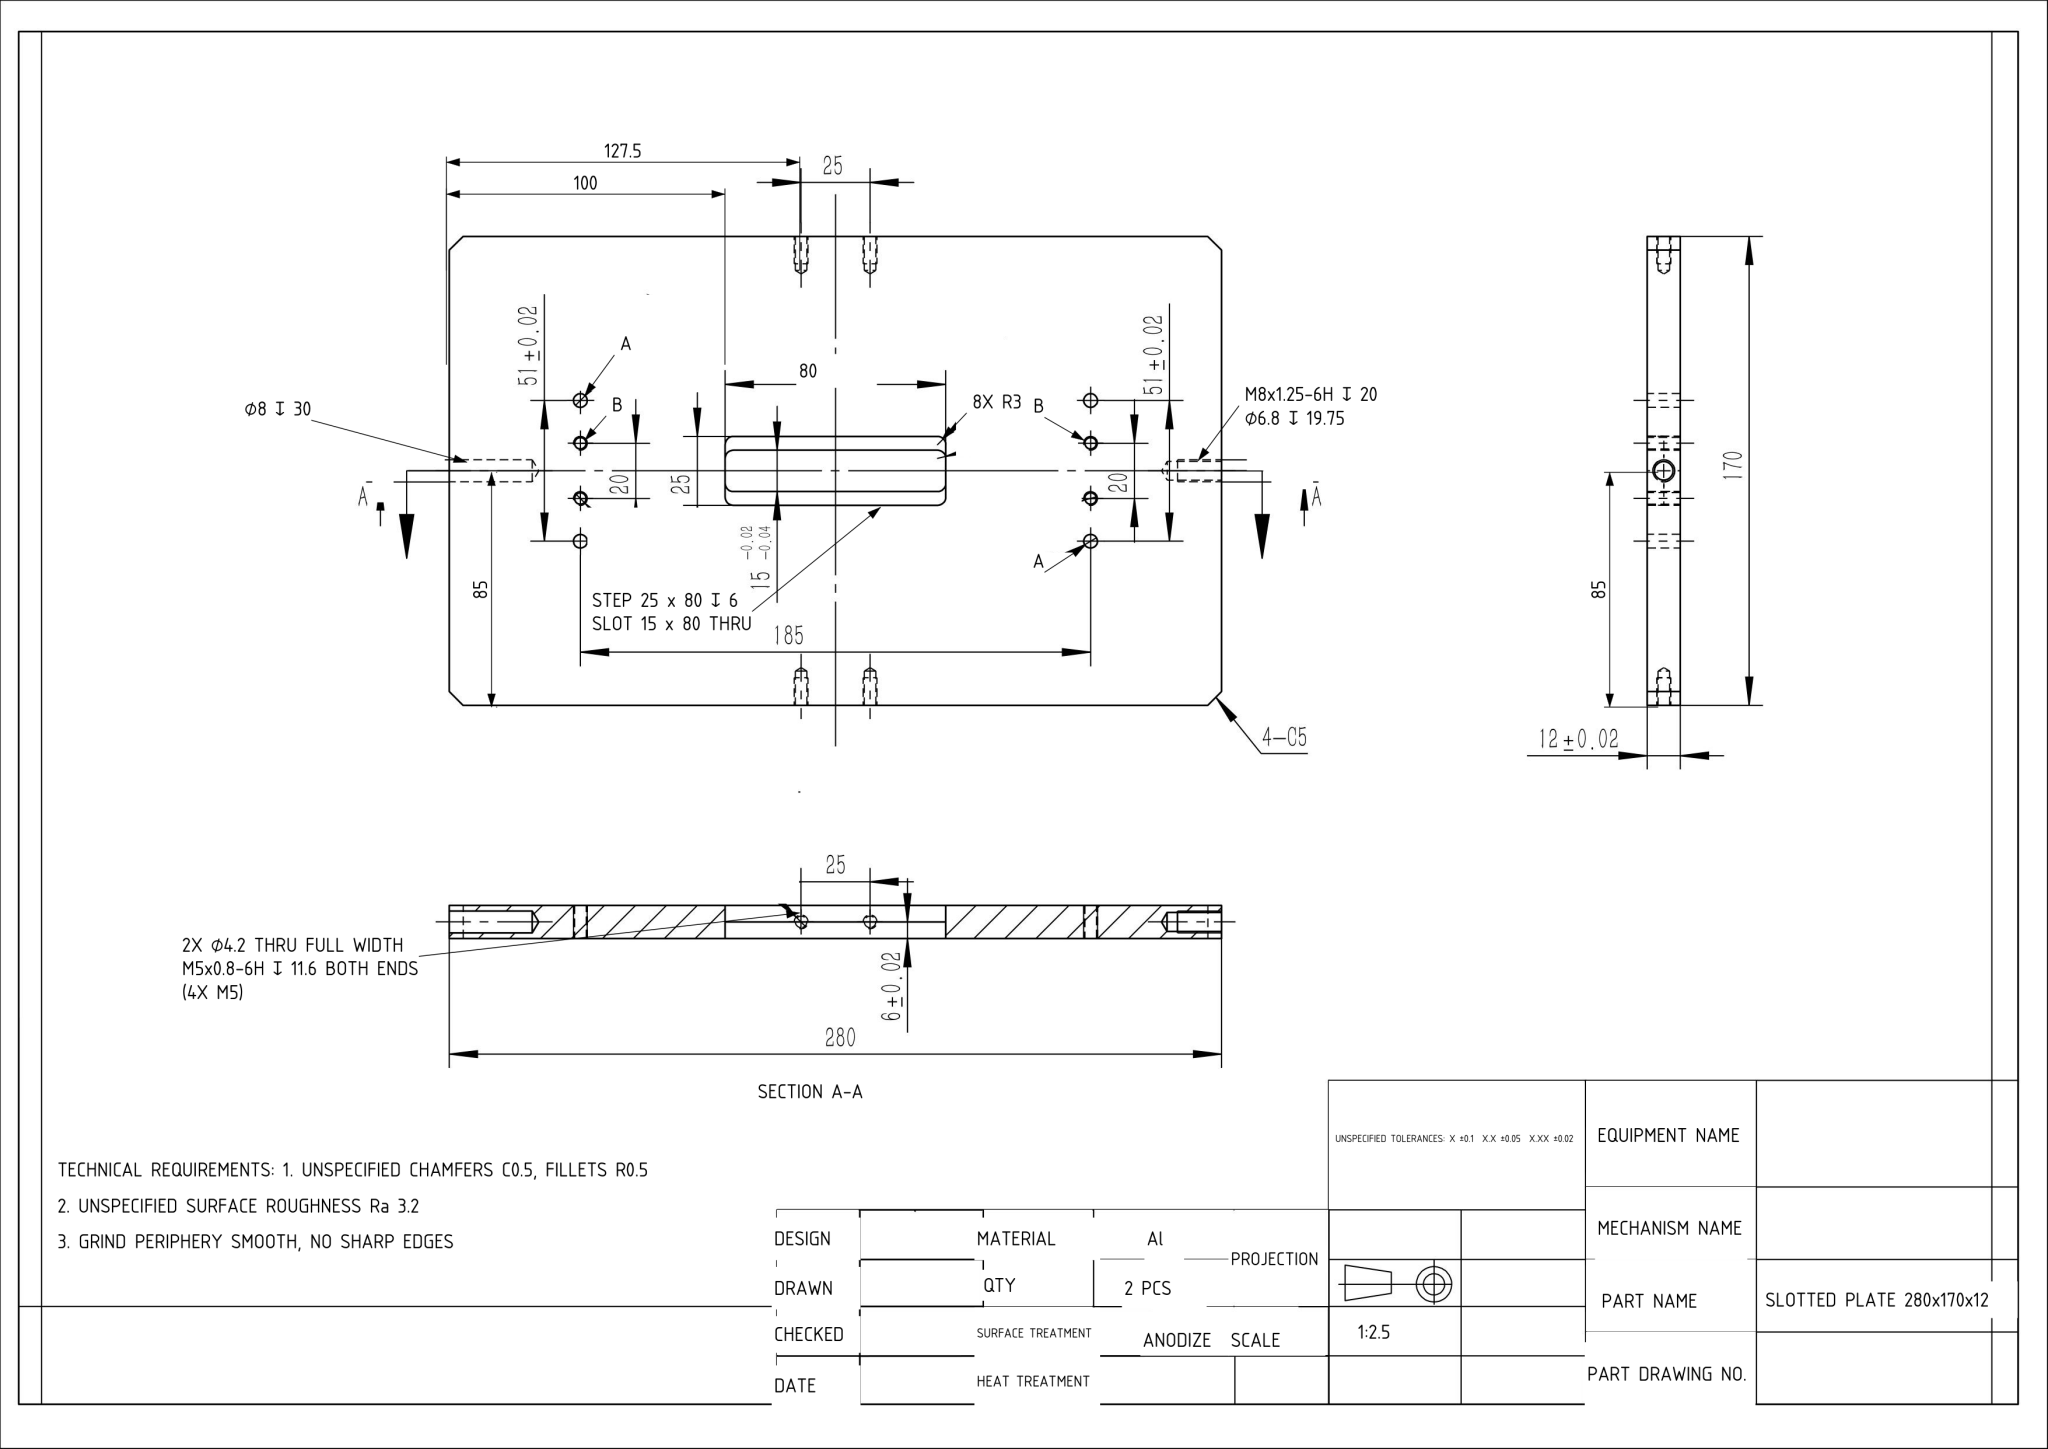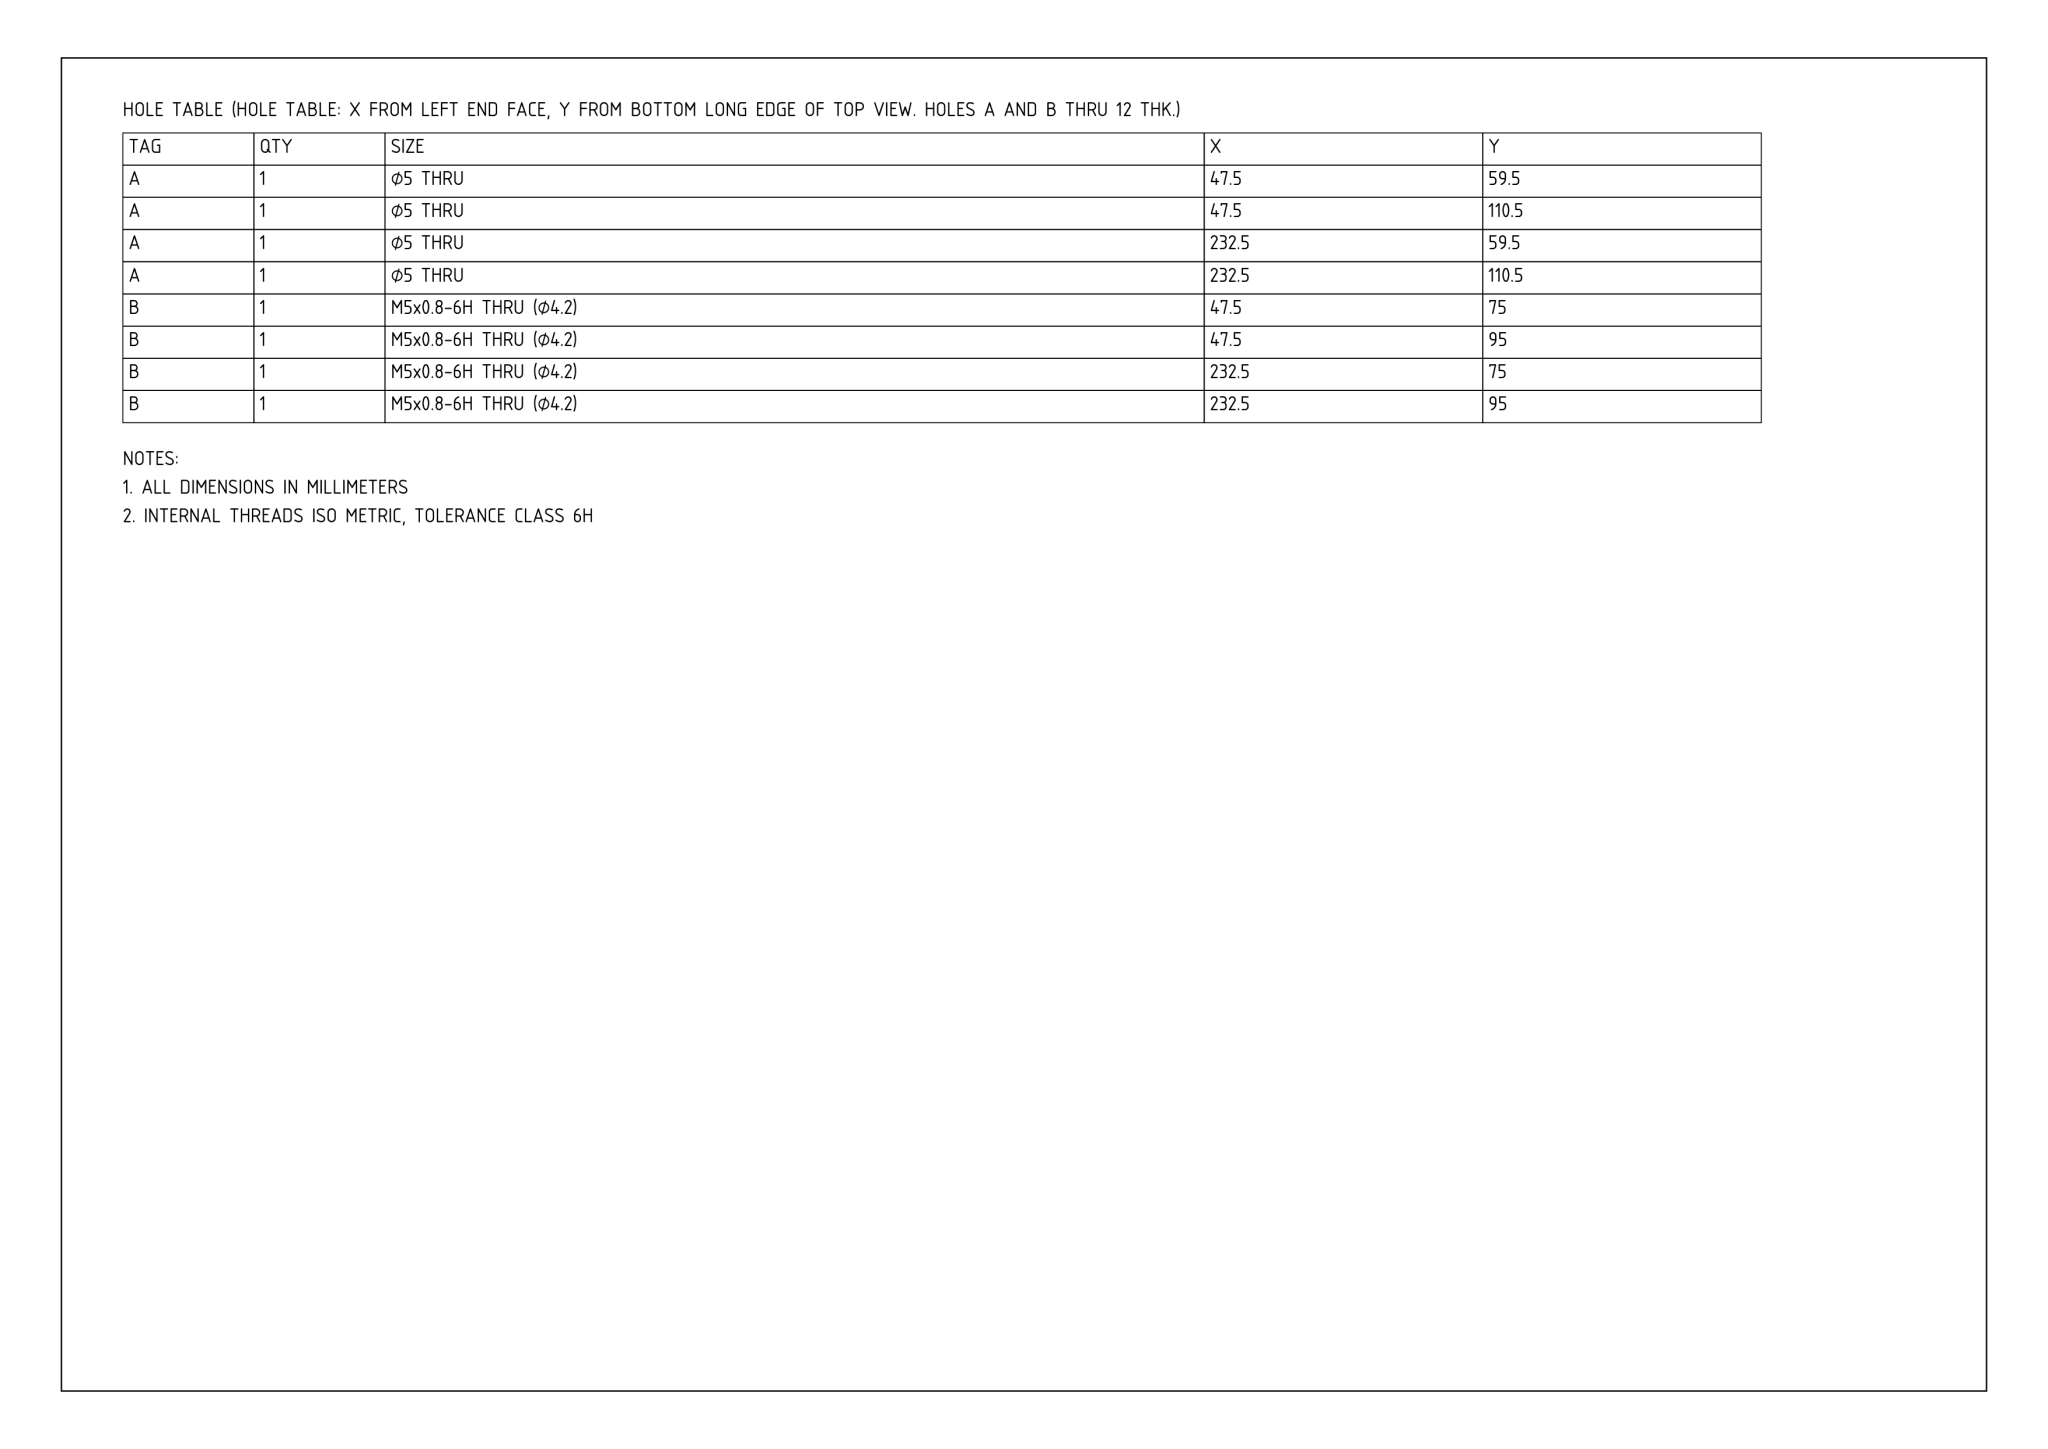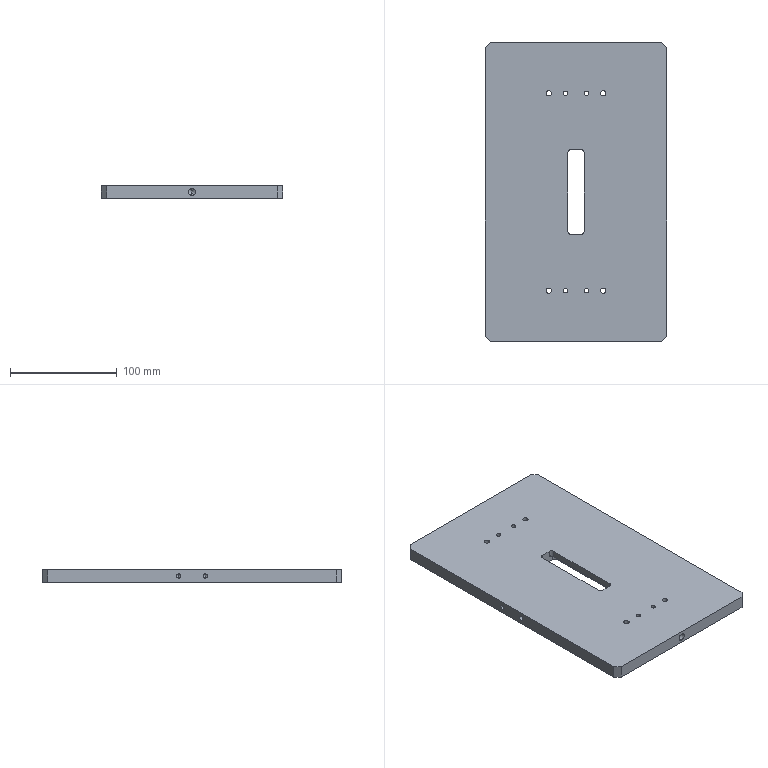Part | NX | mm | 1 solid | 66 faces | box 170 x 280 x 12 mm | volume 546885 mm3 | cylinder 36 | plane 18 | cone 12 | commonest cylinder face diameters 4.2 x16 5 x8 6 x8 8 x2 6.8 x2